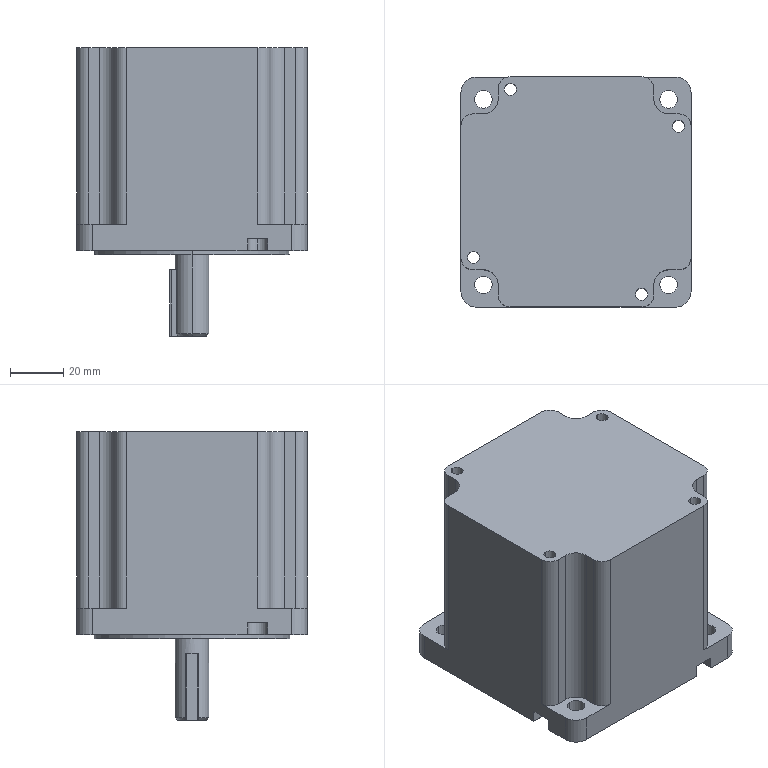Component | SolidWorks | 86StepperMotor-XG2.1-1 | 1 solid | 103 faces | volume 513767 mm3 | plane 44 | cylinder 43 | torus 8 | cone 8 | commonest cylinder face diameters 4.5 x8 6.57 x8 8.9 x8 7.5 x5 11.1 x4 11.4 x4 73 x2 12.7 x2